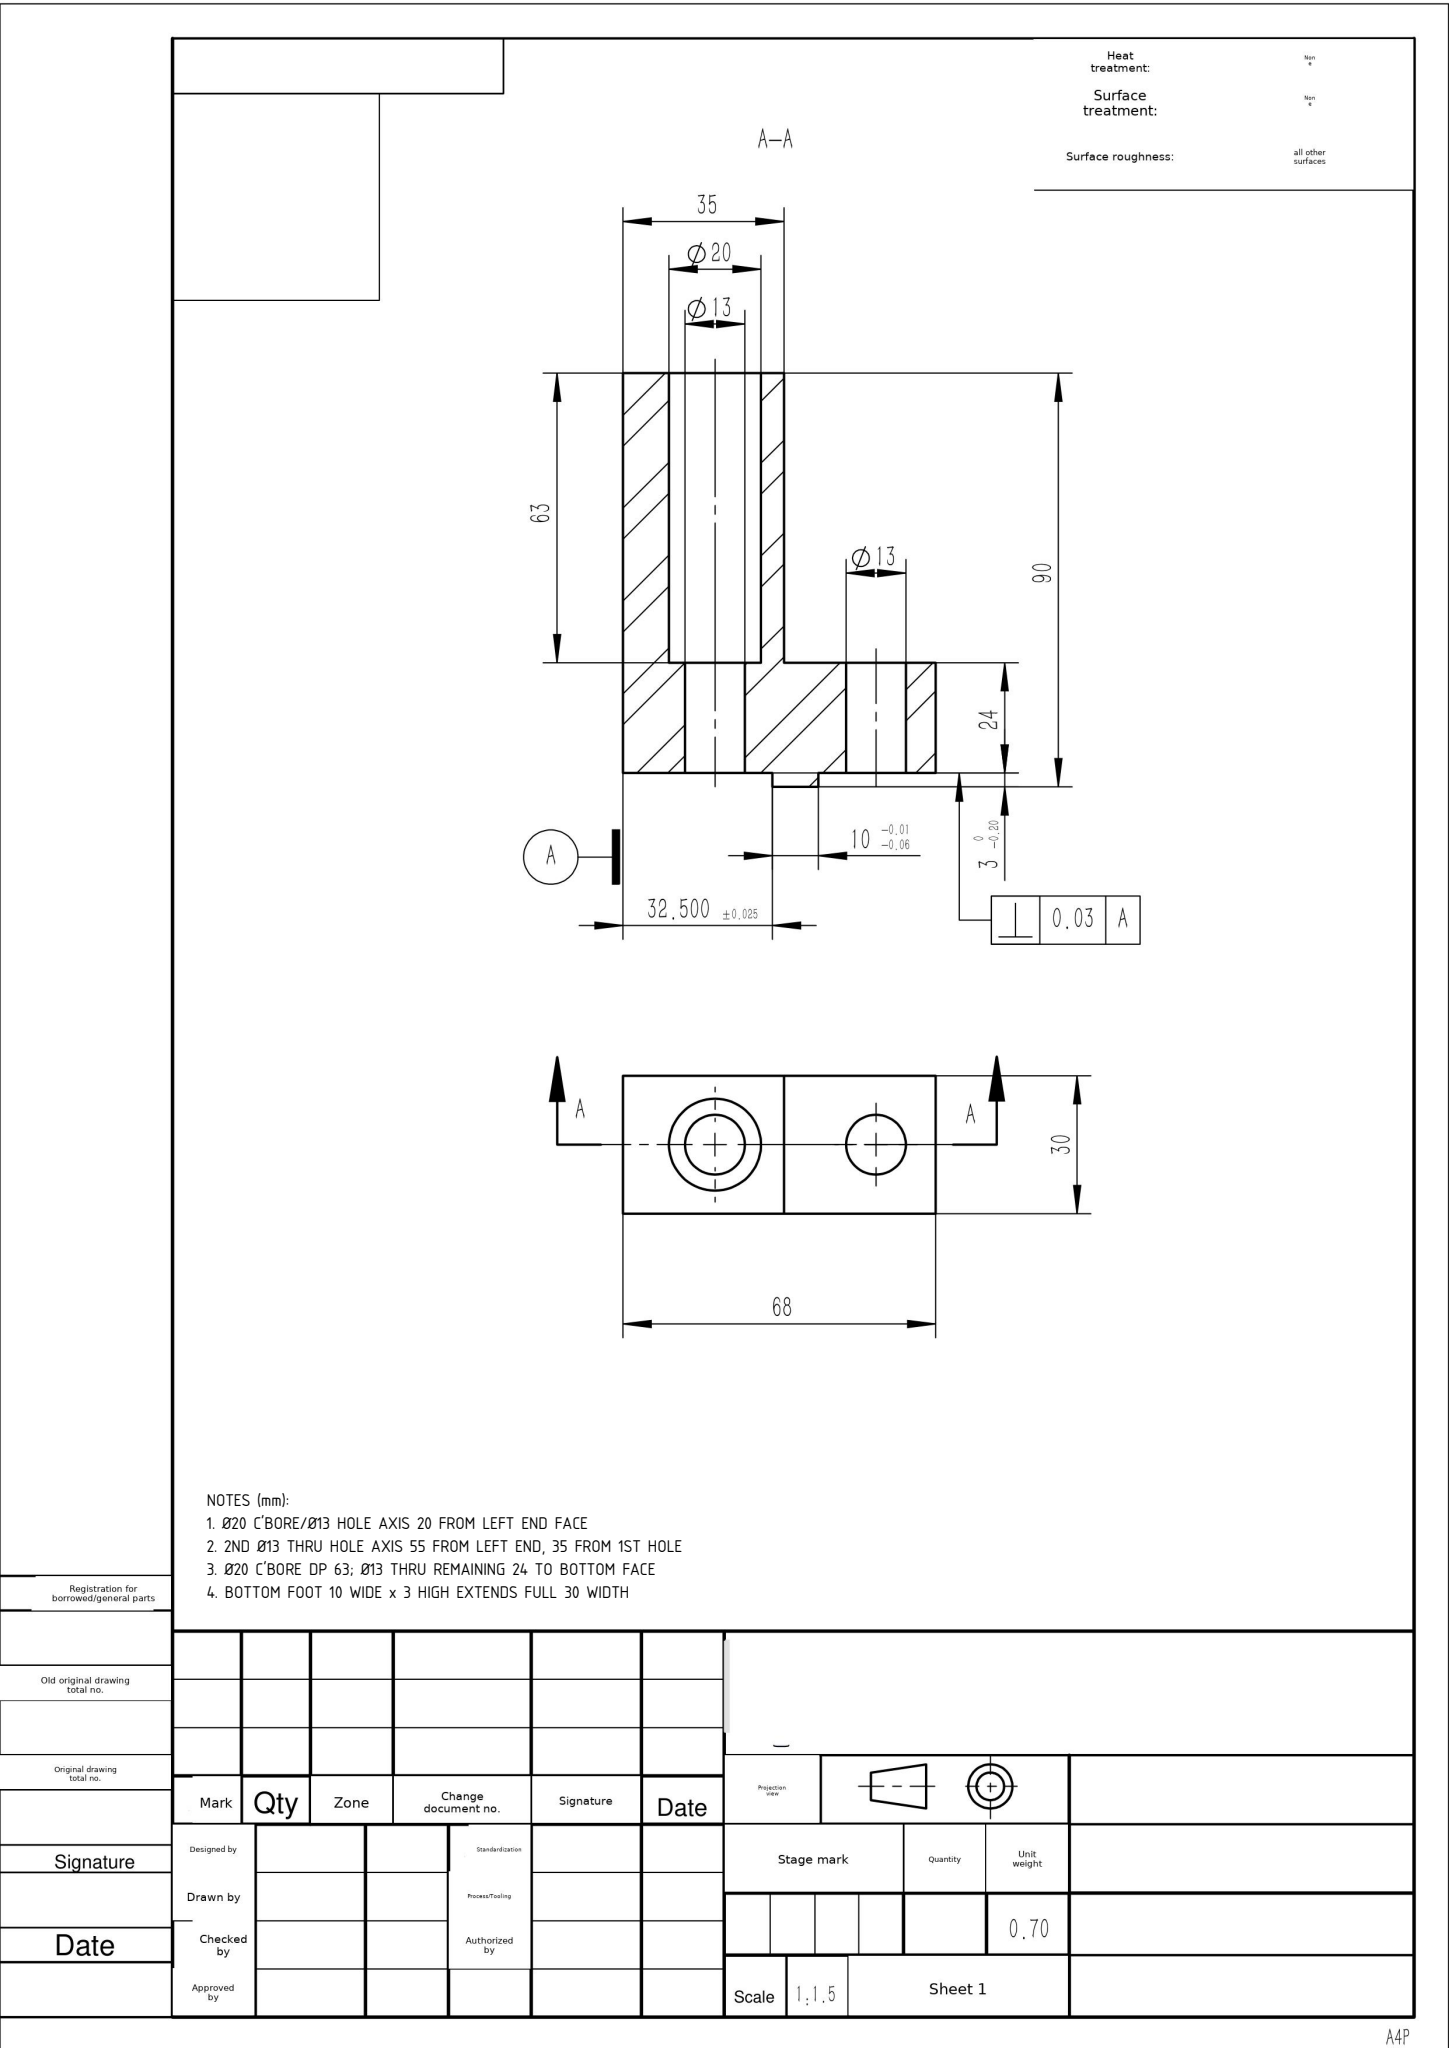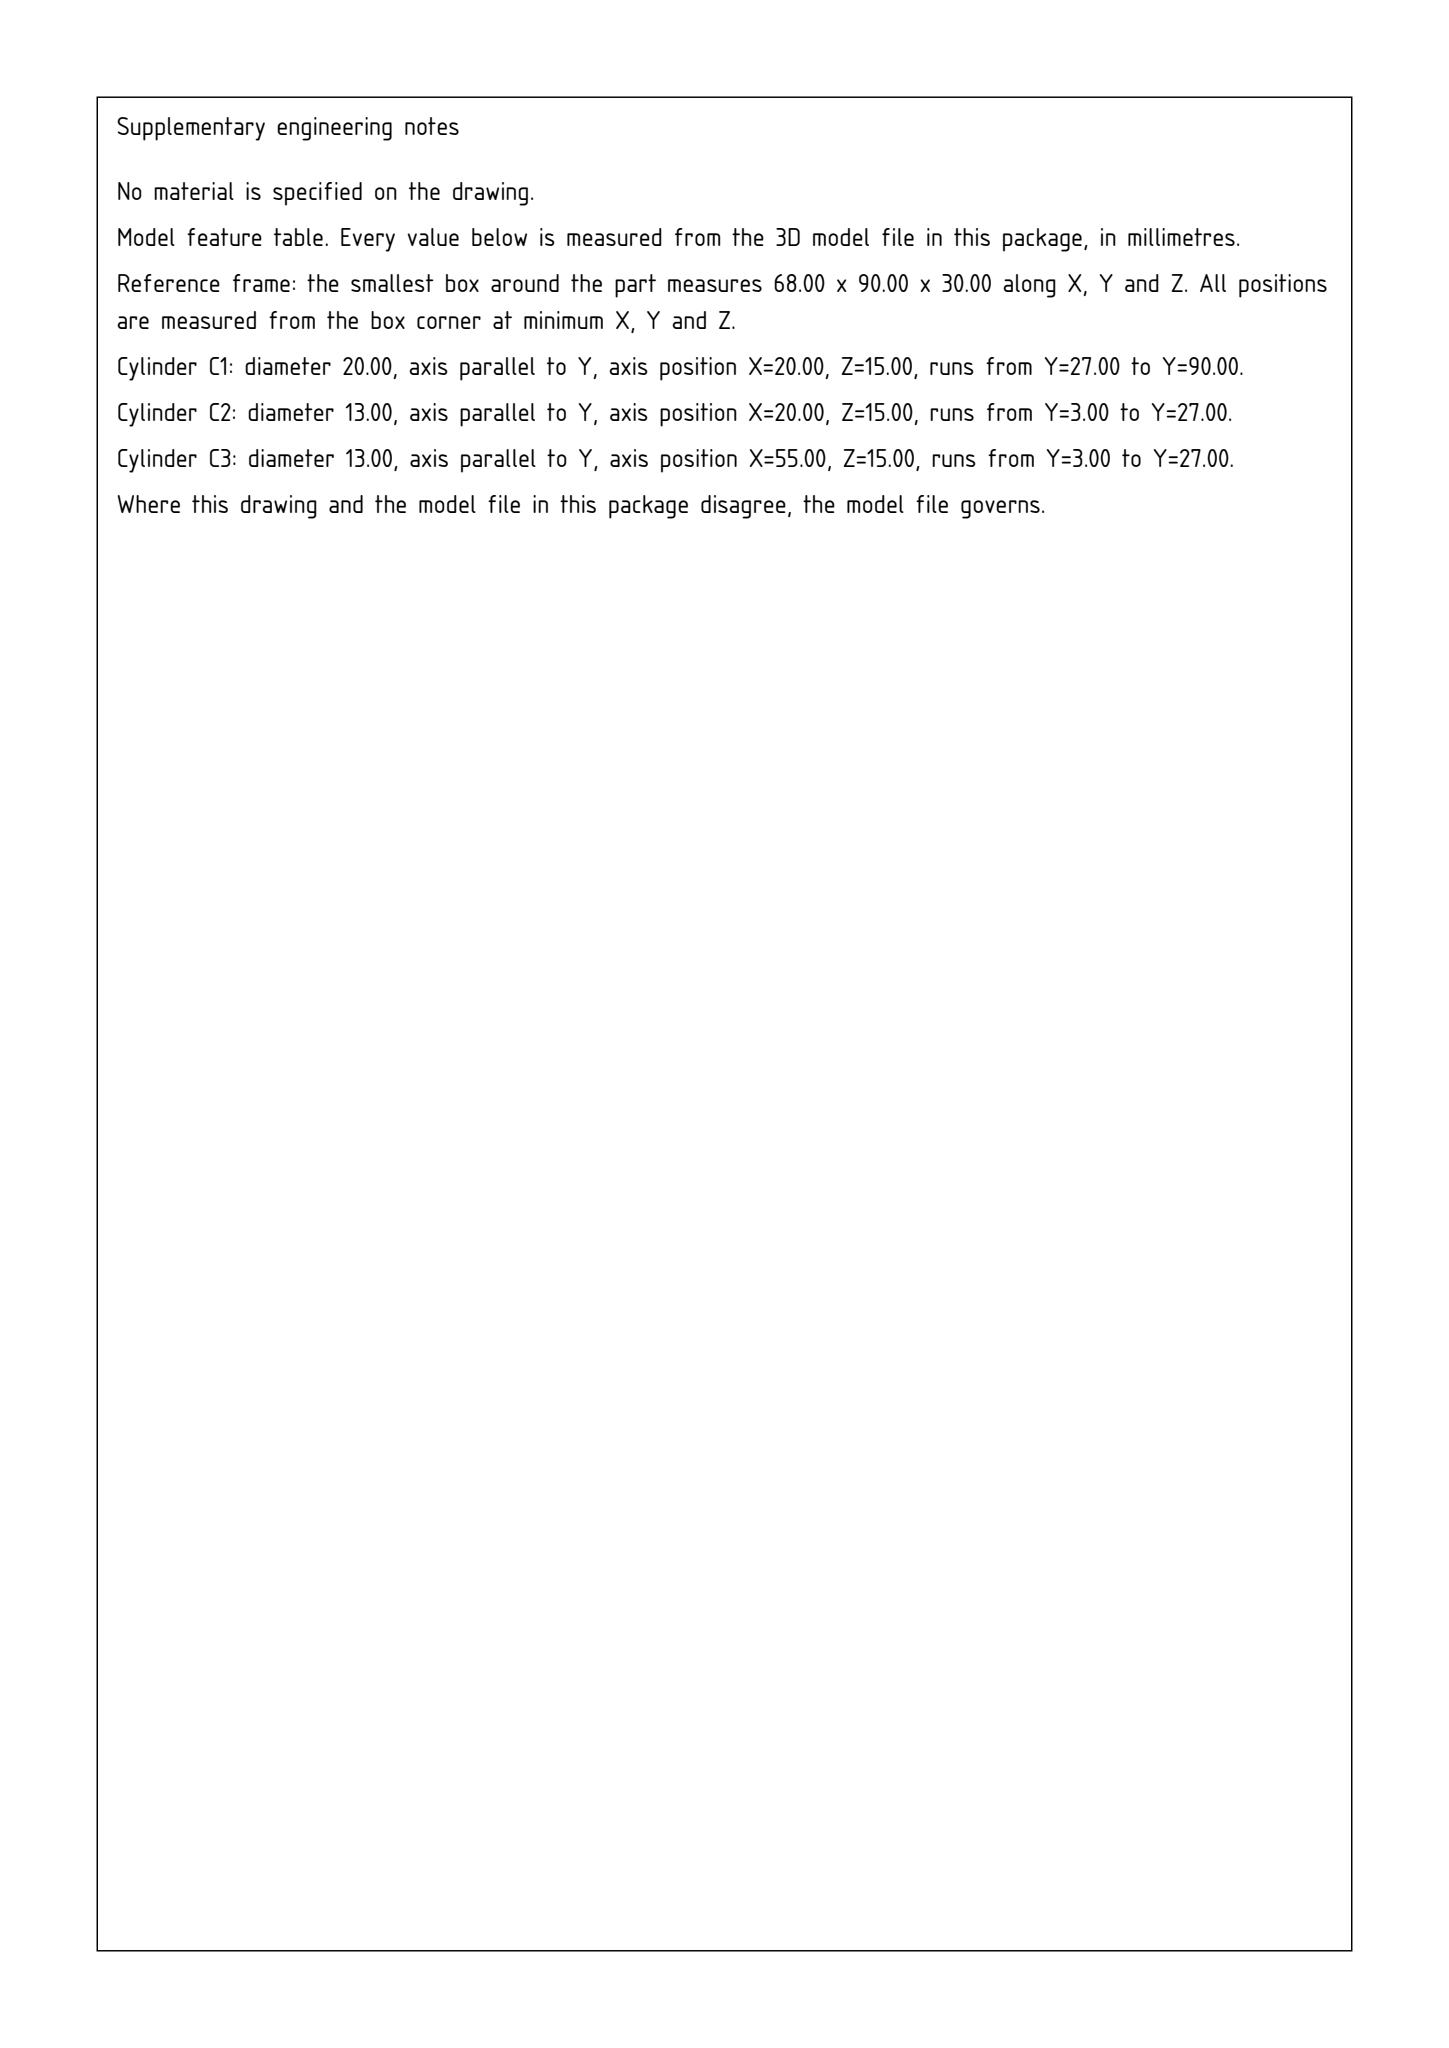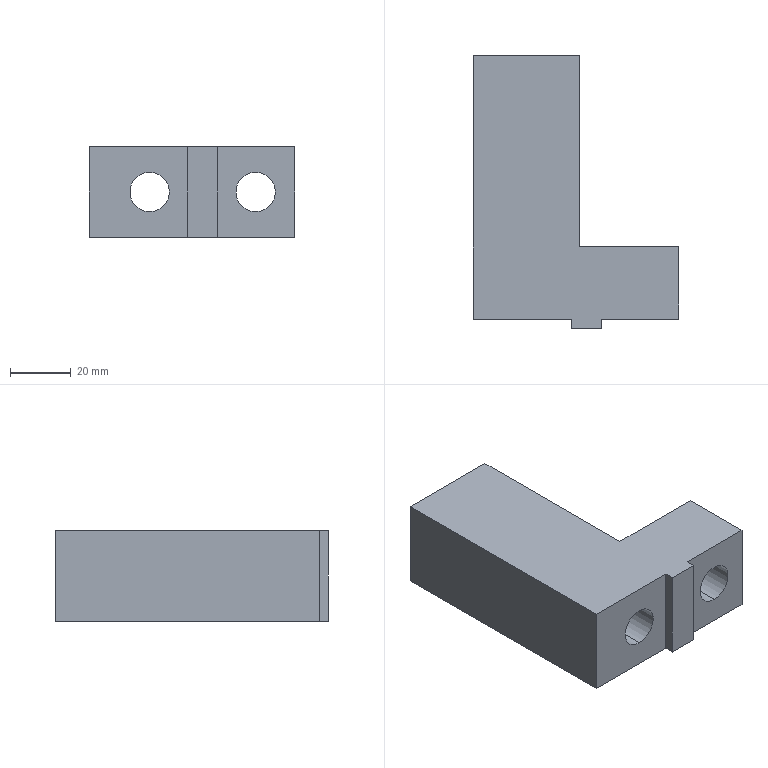Part | SolidWorks | mm | 1 solid | 19 faces | box 68 x 90 x 30 mm | volume 89847 mm3 | plane 13 | cylinder 6 | commonest cylinder face diameters 13 x4 20 x2
Drawing notes:
Ø20 C'BORE/Ø13 HOLE AXIS 20 FROM LEFT END FACE | from the solid: Ø20 & Ø13 cylinders, axis at x=20.0 (bbox x 0-68)
2ND Ø13 THRU HOLE AXIS 55 FROM LEFT END, 35 FROM 1ST HOLE | from the solid: Ø13 cylinder axis at x=55.0; 55-20=35 spacing
Ø20 C'BORE DP 63; Ø13 THRU REMAINING 24 TO BOTTOM FACE | from the solid: Ø20 L=63 (y 27-90), Ø13 L=24 (y 3-27) coaxial at x=20
BOTTOM FOOT 10 WIDE x 3 HIGH EXTENDS FULL 30 WIDTH | from the solid: x-planes 32.5 & 42.5, y-plane 3.0, z-planes 0.0 & 30.0 (bbox z=30)
build123d program:
from build123d import *

# Parameters (mm, degrees)
BOSS_EXTRUDE1_DEPTH = 15
SKETCH2_R           = 6.5
CUT_EXTRUDE1_DEPTH  = 114.794
SKETCH4_W           = 25.5
SKETCH4_H           = 3
SKETCH4_W_2         = 32.5
CUT_EXTRUDE3_DEPTH  = 117.722
SKETCH8_R           = 10
CUT_EXTRUDE6_DEPTH  = 63


with BuildPart() as part:
    # Sketch1 → Boss-Extrude1 (new, symmetric)
    with BuildSketch(Plane.XY):
        Polygon((0, 0), (0, 90), (35, 90), (35, 27), (68, 27), (68, 0), align=None)
    extrude(amount=BOSS_EXTRUDE1_DEPTH, both=True)

    # Sketch2 → Cut-Extrude1 (cut, through all)
    with BuildSketch(Plane(origin=(0, 90, 0), x_dir=(1, 0, 0), z_dir=(0, 1, 0))):
        with Locations(Location((20, 0, 0), (0, 0, 270))):
            Circle(SKETCH2_R)
        with Locations(Location((55, 0, 0), (0, 0, 270))):
            Circle(SKETCH2_R)
    extrude(amount=-CUT_EXTRUDE1_DEPTH, mode=Mode.SUBTRACT)

    # Sketch4 → Cut-Extrude3 (cut, through all)
    with BuildSketch(Plane.XY.offset(15)):
        with Locations((55.25, 1.5)):
            Rectangle(SKETCH4_W, SKETCH4_H)
        with Locations((16.25, 1.5)):
            Rectangle(SKETCH4_W_2, SKETCH4_H)
    extrude(amount=-CUT_EXTRUDE3_DEPTH, mode=Mode.SUBTRACT)

    # Sketch8 → Cut-Extrude6 (cut)
    with BuildSketch(Plane(origin=(0, 90, 0), x_dir=(1, 0, 0), z_dir=(0, 1, 0))):
        with Locations(Location((20, 0, 0), (0, 0, 270))):
            Circle(SKETCH8_R)
    extrude(amount=-CUT_EXTRUDE6_DEPTH, mode=Mode.SUBTRACT)


solid = part.part
STEP:
#1=CARTESIAN_POINT('',(20.,27.,-10.));
#2=VERTEX_POINT('',#1);
#3=CARTESIAN_POINT('',(20.,27.,10.));
#4=VERTEX_POINT('',#3);
#5=CARTESIAN_POINT('',(20.,27.,0.));
#6=DIRECTION('',(0.,1.,0.));
#7=DIRECTION('',(0.,0.,-1.));
#8=AXIS2_PLACEMENT_3D('',#5,#6,#7);
#9=CIRCLE('',#8,10.);
#10=EDGE_CURVE('',#2,#4,#9,.T.);
#11=ORIENTED_EDGE('',*,*,#10,.F.);
#12=CARTESIAN_POINT('',(20.,90.,-10.));
#13=VERTEX_POINT('',#12);
#14=CARTESIAN_POINT('',(20.,-1.284,-10.));
#15=DIRECTION('',(0.,1.,0.));
#16=VECTOR('',#15,1000.);
#17=LINE('',#14,#16);
#18=EDGE_CURVE('',#2,#13,#17,.T.);
#19=ORIENTED_EDGE('',*,*,#18,.T.);
#20=CARTESIAN_POINT('',(20.,90.,10.));
#21=VERTEX_POINT('',#20);
#22=CARTESIAN_POINT('',(20.,90.,0.));
#23=DIRECTION('',(0.,1.,0.));
#24=DIRECTION('',(0.,0.,1.));
#25=AXIS2_PLACEMENT_3D('',#22,#23,#24);
#26=CIRCLE('',#25,10.);
#27=EDGE_CURVE('',#13,#21,#26,.T.);
#28=ORIENTED_EDGE('',*,*,#27,.T.);
#29=CARTESIAN_POINT('',(20.,-1.284,10.));
#30=DIRECTION('',(0.,1.,0.));
#31=VECTOR('',#30,1000.);
#32=LINE('',#29,#31);
#33=EDGE_CURVE('',#4,#21,#32,.T.);
#34=ORIENTED_EDGE('',*,*,#33,.F.);
#35=EDGE_LOOP('',(#11,#19,#28,#34));
#36=FACE_OUTER_BOUND('',#35,.T.);
#37=CARTESIAN_POINT('',(20.,-1.284,0.));
#38=DIRECTION('',(0.,1.,0.));
#39=DIRECTION('',(0.,0.,1.));
#40=AXIS2_PLACEMENT_3D('',#37,#38,#39);
#41=CYLINDRICAL_SURFACE('',#40,10.);
#42=ADVANCED_FACE('',(#36),#41,.F.);
#43=CARTESIAN_POINT('',(55.,3.,6.5));
#44=VERTEX_POINT('',#43);
#45=CARTESIAN_POINT('',(55.,3.,-6.5));
#46=VERTEX_POINT('',#45);
#47=CARTESIAN_POINT('',(55.,3.,0.));
#48=DIRECTION('',(0.,-1.,0.));
#49=DIRECTION('',(-1.,-0.,0.));
#50=AXIS2_PLACEMENT_3D('',#47,#48,#49);
#51=CIRCLE('',#50,6.5);
#52=EDGE_CURVE('',#44,#46,#51,.T.);
#53=ORIENTED_EDGE('',*,*,#52,.T.);
#54=CARTESIAN_POINT('',(55.,27.,-6.5));
#55=VERTEX_POINT('',#54);
#56=CARTESIAN_POINT('',(55.,0.,-6.5));
#57=DIRECTION('',(0.,1.,0.));
#58=VECTOR('',#57,1000.);
#59=LINE('',#56,#58);
#60=EDGE_CURVE('',#46,#55,#59,.T.);
#61=ORIENTED_EDGE('',*,*,#60,.T.);
#62=CARTESIAN_POINT('',(55.,27.,6.5));
#63=VERTEX_POINT('',#62);
#64=CARTESIAN_POINT('',(55.,27.,0.));
#65=DIRECTION('',(0.,-1.,0.));
#66=DIRECTION('',(0.,0.,-1.));
#67=AXIS2_PLACEMENT_3D('',#64,#65,#66);
#68=CIRCLE('',#67,6.5);
#69=EDGE_CURVE('',#63,#55,#68,.T.);
#70=ORIENTED_EDGE('',*,*,#69,.F.);
#71=CARTESIAN_POINT('',(55.,0.,6.5));
#72=DIRECTION('',(0.,1.,0.));
#73=VECTOR('',#72,1000.);
#74=LINE('',#71,#73);
#75=EDGE_CURVE('',#44,#63,#74,.T.);
#76=ORIENTED_EDGE('',*,*,#75,.F.);
#77=EDGE_LOOP('',(#53,#61,#70,#76));
#78=FACE_OUTER_BOUND('',#77,.T.);
#79=CARTESIAN_POINT('',(55.,0.,0.));
#80=DIRECTION('',(0.,1.,0.));
#81=DIRECTION('',(0.,0.,1.));
#82=AXIS2_PLACEMENT_3D('',#79,#80,#81);
#83=CYLINDRICAL_SURFACE('',#82,6.5);
#84=ADVANCED_FACE('',(#78),#83,.F.);
#85=CARTESIAN_POINT('',(20.,3.,6.5));
#86=VERTEX_POINT('',#85);
#87=CARTESIAN_POINT('',(20.,3.,-6.5));
#88=VERTEX_POINT('',#87);
#89=CARTESIAN_POINT('',(20.,3.,0.));
#90=DIRECTION('',(0.,-1.,0.));
#91=DIRECTION('',(-1.,-0.,0.));
#92=AXIS2_PLACEMENT_3D('',#89,#90,#91);
#93=CIRCLE('',#92,6.5);
#94=EDGE_CURVE('',#86,#88,#93,.T.);
#95=ORIENTED_EDGE('',*,*,#94,.T.);
#96=CARTESIAN_POINT('',(20.,27.,-6.5));
#97=VERTEX_POINT('',#96);
#98=CARTESIAN_POINT('',(20.,0.,-6.5));
#99=DIRECTION('',(0.,1.,0.));
#100=VECTOR('',#99,1000.);
#101=LINE('',#98,#100);
#102=EDGE_CURVE('',#88,#97,#101,.T.);
#103=ORIENTED_EDGE('',*,*,#102,.T.);
#104=CARTESIAN_POINT('',(20.,27.,6.5));
#105=VERTEX_POINT('',#104);
#106=CARTESIAN_POINT('',(20.,27.,0.));
#107=DIRECTION('',(0.,1.,0.));
#108=DIRECTION('',(0.,0.,-1.));
#109=AXIS2_PLACEMENT_3D('',#106,#107,#108);
#110=CIRCLE('',#109,6.5);
#111=EDGE_CURVE('',#97,#105,#110,.T.);
#112=ORIENTED_EDGE('',*,*,#111,.T.);
#113=CARTESIAN_POINT('',(20.,0.,6.5));
#114=DIRECTION('',(0.,1.,0.));
#115=VECTOR('',#114,1000.);
#116=LINE('',#113,#115);
#117=EDGE_CURVE('',#86,#105,#116,.T.);
#118=ORIENTED_EDGE('',*,*,#117,.F.);
#119=EDGE_LOOP('',(#95,#103,#112,#118));
#120=FACE_OUTER_BOUND('',#119,.T.);
#121=CARTESIAN_POINT('',(20.,0.,0.));
#122=DIRECTION('',(0.,1.,0.));
#123=DIRECTION('',(0.,0.,1.));
#124=AXIS2_PLACEMENT_3D('',#121,#122,#123);
#125=CYLINDRICAL_SURFACE('',#124,6.5);
#126=ADVANCED_FACE('',(#120),#125,.F.);
#127=CARTESIAN_POINT('',(32.5,0.,15.));
#128=VERTEX_POINT('',#127);
#129=CARTESIAN_POINT('',(42.5,-0.,15.));
#130=VERTEX_POINT('',#129);
#131=CARTESIAN_POINT('',(68.,-0.,15.));
#132=DIRECTION('',(1.,-0.,0.));
#133=VECTOR('',#132,1000.);
#134=LINE('',#131,#133);
#135=EDGE_CURVE('',#128,#130,#134,.T.);
#136=ORIENTED_EDGE('',*,*,#135,.F.);
#137=CARTESIAN_POINT('',(32.5,0.,-15.));
#138=VERTEX_POINT('',#137);
#139=CARTESIAN_POINT('',(32.5,0.,-15.));
#140=DIRECTION('',(0.,0.,1.));
#141=VECTOR('',#140,1000.);
#142=LINE('',#139,#141);
#143=EDGE_CURVE('',#138,#128,#142,.T.);
#144=ORIENTED_EDGE('',*,*,#143,.F.);
#145=CARTESIAN_POINT('',(42.5,-0.,-15.));
#146=VERTEX_POINT('',#145);
#147=CARTESIAN_POINT('',(68.,-0.,-15.));
#148=DIRECTION('',(1.,-0.,0.));
#149=VECTOR('',#148,1000.);
#150=LINE('',#147,#149);
#151=EDGE_CURVE('',#138,#146,#150,.T.);
#152=ORIENTED_EDGE('',*,*,#151,.T.);
#153=CARTESIAN_POINT('',(42.5,-0.,-15.));
#154=DIRECTION('',(0.,0.,1.));
#155=VECTOR('',#154,1000.);
#156=LINE('',#153,#155);
#157=EDGE_CURVE('',#146,#130,#156,.T.);
#158=ORIENTED_EDGE('',*,*,#157,.T.);
#159=EDGE_LOOP('',(#136,#144,#152,#158));
#160=FACE_OUTER_BOUND('',#159,.T.);
#161=CARTESIAN_POINT('',(68.,-0.,15.));
#162=DIRECTION('',(0.,1.,0.));
#163=DIRECTION('',(-1.,0.,0.));
#164=AXIS2_PLACEMENT_3D('',#161,#162,#163);
#165=PLANE('',#164);
#166=ADVANCED_FACE('',(#160),#165,.F.);
#167=CARTESIAN_POINT('',(68.,3.,15.));
#168=VERTEX_POINT('',#167);
#169=CARTESIAN_POINT('',(68.,27.,15.));
#170=VERTEX_POINT('',#169);
#171=CARTESIAN_POINT('',(68.,27.,15.));
#172=DIRECTION('',(0.,1.,0.));
#173=VECTOR('',#172,1000.);
#174=LINE('',#171,#173);
#175=EDGE_CURVE('',#168,#170,#174,.T.);
#176=ORIENTED_EDGE('',*,*,#175,.F.);
#177=CARTESIAN_POINT('',(68.,3.,-15.));
#178=VERTEX_POINT('',#177);
#179=CARTESIAN_POINT('',(68.,3.,-15.));
#180=DIRECTION('',(0.,0.,1.));
#181=VECTOR('',#180,1000.);
#182=LINE('',#179,#181);
#183=EDGE_CURVE('',#178,#168,#182,.T.);
#184=ORIENTED_EDGE('',*,*,#183,.F.);
#185=CARTESIAN_POINT('',(68.,27.,-15.));
#186=VERTEX_POINT('',#185);
#187=CARTESIAN_POINT('',(68.,27.,-15.));
#188=DIRECTION('',(0.,1.,0.));
#189=VECTOR('',#188,1000.);
#190=LINE('',#187,#189);
#191=EDGE_CURVE('',#178,#186,#190,.T.);
#192=ORIENTED_EDGE('',*,*,#191,.T.);
#193=CARTESIAN_POINT('',(68.,27.,15.));
#194=DIRECTION('',(0.,0.,-1.));
#195=VECTOR('',#194,1000.);
#196=LINE('',#193,#195);
#197=EDGE_CURVE('',#170,#186,#196,.T.);
#198=ORIENTED_EDGE('',*,*,#197,.F.);
#199=EDGE_LOOP('',(#176,#184,#192,#198));
#200=FACE_OUTER_BOUND('',#199,.T.);
#201=CARTESIAN_POINT('',(68.,27.,15.));
#202=DIRECTION('',(-1.,0.,0.));
#203=DIRECTION('',(0.,0.,1.));
#204=AXIS2_PLACEMENT_3D('',#201,#202,#203);
#205=PLANE('',#204);
#206=ADVANCED_FACE('',(#200),#205,.F.);
#207=ORIENTED_EDGE('',*,*,#69,.T.);
#208=CARTESIAN_POINT('',(55.,27.,0.));
#209=DIRECTION('',(0.,-1.,0.));
#210=DIRECTION('',(0.,0.,-1.));
#211=AXIS2_PLACEMENT_3D('',#208,#209,#210);
#212=CIRCLE('',#211,6.5);
#213=EDGE_CURVE('',#55,#63,#212,.T.);
#214=ORIENTED_EDGE('',*,*,#213,.T.);
#215=EDGE_LOOP('',(#207,#214));
#216=FACE_BOUND('',#215,.T.);
#217=CARTESIAN_POINT('',(35.,27.,-15.));
#218=VERTEX_POINT('',#217);
#219=CARTESIAN_POINT('',(35.,27.,-15.));
#220=DIRECTION('',(-1.,0.,0.));
#221=VECTOR('',#220,1000.);
#222=LINE('',#219,#221);
#223=EDGE_CURVE('',#186,#218,#222,.T.);
#224=ORIENTED_EDGE('',*,*,#223,.T.);
#225=CARTESIAN_POINT('',(35.,27.,15.));
#226=VERTEX_POINT('',#225);
#227=CARTESIAN_POINT('',(35.,27.,15.));
#228=DIRECTION('',(0.,0.,-1.));
#229=VECTOR('',#228,1000.);
#230=LINE('',#227,#229);
#231=EDGE_CURVE('',#226,#218,#230,.T.);
#232=ORIENTED_EDGE('',*,*,#231,.F.);
#233=CARTESIAN_POINT('',(35.,27.,15.));
#234=DIRECTION('',(-1.,0.,0.));
#235=VECTOR('',#234,1000.);
#236=LINE('',#233,#235);
#237=EDGE_CURVE('',#170,#226,#236,.T.);
#238=ORIENTED_EDGE('',*,*,#237,.F.);
#239=ORIENTED_EDGE('',*,*,#197,.T.);
#240=EDGE_LOOP('',(#224,#232,#238,#239));
#241=FACE_OUTER_BOUND('',#240,.T.);
#242=CARTESIAN_POINT('',(35.,27.,15.));
#243=DIRECTION('',(0.,-1.,0.));
#244=DIRECTION('',(0.,0.,-1.));
#245=AXIS2_PLACEMENT_3D('',#242,#243,#244);
#246=PLANE('',#245);
#247=ADVANCED_FACE('',(#216,#241),#246,.F.);
#248=CARTESIAN_POINT('',(35.,90.,-15.));
#249=VERTEX_POINT('',#248);
#250=CARTESIAN_POINT('',(35.,90.,-15.));
#251=DIRECTION('',(-0.,1.,0.));
#252=VECTOR('',#251,1000.);
#253=LINE('',#250,#252);
#254=EDGE_CURVE('',#218,#249,#253,.T.);
#255=ORIENTED_EDGE('',*,*,#254,.T.);
#256=CARTESIAN_POINT('',(35.,90.,15.));
#257=VERTEX_POINT('',#256);
#258=CARTESIAN_POINT('',(35.,90.,15.));
#259=DIRECTION('',(0.,0.,-1.));
#260=VECTOR('',#259,1000.);
#261=LINE('',#258,#260);
#262=EDGE_CURVE('',#257,#249,#261,.T.);
#263=ORIENTED_EDGE('',*,*,#262,.F.);
#264=CARTESIAN_POINT('',(35.,90.,15.));
#265=DIRECTION('',(-0.,1.,0.));
#266=VECTOR('',#265,1000.);
#267=LINE('',#264,#266);
#268=EDGE_CURVE('',#226,#257,#267,.T.);
#269=ORIENTED_EDGE('',*,*,#268,.F.);
#270=ORIENTED_EDGE('',*,*,#231,.T.);
#271=EDGE_LOOP('',(#255,#263,#269,#270));
#272=FACE_OUTER_BOUND('',#271,.T.);
#273=CARTESIAN_POINT('',(35.,90.,15.));
#274=DIRECTION('',(-1.,-0.,0.));
#275=DIRECTION('',(0.,-1.,0.));
#276=AXIS2_PLACEMENT_3D('',#273,#274,#275);
#277=PLANE('',#276);
#278=ADVANCED_FACE('',(#272),#277,.F.);
#279=CARTESIAN_POINT('',(20.,90.,0.));
#280=DIRECTION('',(0.,1.,0.));
#281=DIRECTION('',(0.,0.,1.));
#282=AXIS2_PLACEMENT_3D('',#279,#280,#281);
#283=CIRCLE('',#282,10.);
#284=EDGE_CURVE('',#21,#13,#283,.T.);
#285=ORIENTED_EDGE('',*,*,#284,.F.);
#286=ORIENTED_EDGE('',*,*,#27,.F.);
#287=EDGE_LOOP('',(#285,#286));
#288=FACE_BOUND('',#287,.T.);
#289=CARTESIAN_POINT('',(0.,90.,-15.));
#290=VERTEX_POINT('',#289);
#291=CARTESIAN_POINT('',(0.,90.,-15.));
#292=DIRECTION('',(-1.,0.,0.));
#293=VECTOR('',#292,1000.);
#294=LINE('',#291,#293);
#295=EDGE_CURVE('',#249,#290,#294,.T.);
#296=ORIENTED_EDGE('',*,*,#295,.T.);
#297=CARTESIAN_POINT('',(0.,90.,15.));
#298=VERTEX_POINT('',#297);
#299=CARTESIAN_POINT('',(0.,90.,15.));
#300=DIRECTION('',(0.,0.,-1.));
#301=VECTOR('',#300,1000.);
#302=LINE('',#299,#301);
#303=EDGE_CURVE('',#298,#290,#302,.T.);
#304=ORIENTED_EDGE('',*,*,#303,.F.);
#305=CARTESIAN_POINT('',(0.,90.,15.));
#306=DIRECTION('',(-1.,0.,0.));
#307=VECTOR('',#306,1000.);
#308=LINE('',#305,#307);
#309=EDGE_CURVE('',#257,#298,#308,.T.);
#310=ORIENTED_EDGE('',*,*,#309,.F.);
#311=ORIENTED_EDGE('',*,*,#262,.T.);
#312=EDGE_LOOP('',(#296,#304,#310,#311));
#313=FACE_OUTER_BOUND('',#312,.T.);
#314=CARTESIAN_POINT('',(0.,90.,15.));
#315=DIRECTION('',(0.,-1.,0.));
#316=DIRECTION('',(0.,0.,-1.));
#317=AXIS2_PLACEMENT_3D('',#314,#315,#316);
#318=PLANE('',#317);
#319=ADVANCED_FACE('',(#288,#313),#318,.F.);
#320=CARTESIAN_POINT('',(0.,3.,-15.));
#321=VERTEX_POINT('',#320);
#322=CARTESIAN_POINT('',(0.,0.,-15.));
#323=DIRECTION('',(0.,-1.,0.));
#324=VECTOR('',#323,1000.);
#325=LINE('',#322,#324);
#326=EDGE_CURVE('',#290,#321,#325,.T.);
#327=ORIENTED_EDGE('',*,*,#326,.T.);
#328=CARTESIAN_POINT('',(0.,3.,15.));
#329=VERTEX_POINT('',#328);
#330=CARTESIAN_POINT('',(0.,3.,-15.));
#331=DIRECTION('',(0.,0.,1.));
#332=VECTOR('',#331,1000.);
#333=LINE('',#330,#332);
#334=EDGE_CURVE('',#321,#329,#333,.T.);
#335=ORIENTED_EDGE('',*,*,#334,.T.);
#336=CARTESIAN_POINT('',(0.,0.,15.));
#337=DIRECTION('',(0.,-1.,0.));
#338=VECTOR('',#337,1000.);
#339=LINE('',#336,#338);
#340=EDGE_CURVE('',#298,#329,#339,.T.);
#341=ORIENTED_EDGE('',*,*,#340,.F.);
#342=ORIENTED_EDGE('',*,*,#303,.T.);
#343=EDGE_LOOP('',(#327,#335,#341,#342));
#344=FACE_OUTER_BOUND('',#343,.T.);
#345=CARTESIAN_POINT('',(0.,0.,15.));
#346=DIRECTION('',(1.,0.,0.));
#347=DIRECTION('',(0.,0.,-1.));
#348=AXIS2_PLACEMENT_3D('',#345,#346,#347);
#349=PLANE('',#348);
#350=ADVANCED_FACE('',(#344),#349,.F.);
#351=ORIENTED_EDGE('',*,*,#340,.T.);
#352=CARTESIAN_POINT('',(32.5,3.,15.));
#353=VERTEX_POINT('',#352);
#354=CARTESIAN_POINT('',(0.,3.,15.));
#355=DIRECTION('',(-1.,-0.,0.));
#356=VECTOR('',#355,1000.);
#357=LINE('',#354,#356);
#358=EDGE_CURVE('',#353,#329,#357,.T.);
#359=ORIENTED_EDGE('',*,*,#358,.F.);
#360=CARTESIAN_POINT('',(32.5,0.,15.));
#361=DIRECTION('',(0.,1.,0.));
#362=VECTOR('',#361,1000.);
#363=LINE('',#360,#362);
#364=EDGE_CURVE('',#128,#353,#363,.T.);
#365=ORIENTED_EDGE('',*,*,#364,.F.);
#366=ORIENTED_EDGE('',*,*,#135,.T.);
#367=CARTESIAN_POINT('',(42.5,3.,15.));
#368=VERTEX_POINT('',#367);
#369=CARTESIAN_POINT('',(42.5,-0.,15.));
#370=DIRECTION('',(0.,-1.,0.));
#371=VECTOR('',#370,1000.);
#372=LINE('',#369,#371);
#373=EDGE_CURVE('',#368,#130,#372,.T.);
#374=ORIENTED_EDGE('',*,*,#373,.F.);
#375=CARTESIAN_POINT('',(68.,3.,15.));
#376=DIRECTION('',(-1.,-0.,0.));
#377=VECTOR('',#376,1000.);
#378=LINE('',#375,#377);
#379=EDGE_CURVE('',#168,#368,#378,.T.);
#380=ORIENTED_EDGE('',*,*,#379,.F.);
#381=ORIENTED_EDGE('',*,*,#175,.T.);
#382=ORIENTED_EDGE('',*,*,#237,.T.);
#383=ORIENTED_EDGE('',*,*,#268,.T.);
#384=ORIENTED_EDGE('',*,*,#309,.T.);
#385=EDGE_LOOP('',(#351,#359,#365,#366,#374,#380,#381,#382,#383,#384));
#386=FACE_OUTER_BOUND('',#385,.T.);
#387=CARTESIAN_POINT('',(0.,0.,15.));
#388=DIRECTION('',(0.,0.,-1.));
#389=DIRECTION('',(-1.,0.,0.));
#390=AXIS2_PLACEMENT_3D('',#387,#388,#389);
#391=PLANE('',#390);
#392=ADVANCED_FACE('',(#386),#391,.F.);
#393=CARTESIAN_POINT('',(32.5,3.,-15.));
#394=VERTEX_POINT('',#393);
#395=CARTESIAN_POINT('',(0.,3.,-15.));
#396=DIRECTION('',(-1.,-0.,0.));
#397=VECTOR('',#396,1000.);
#398=LINE('',#395,#397);
#399=EDGE_CURVE('',#394,#321,#398,.T.);
#400=ORIENTED_EDGE('',*,*,#399,.T.);
#401=ORIENTED_EDGE('',*,*,#326,.F.);
#402=ORIENTED_EDGE('',*,*,#295,.F.);
#403=ORIENTED_EDGE('',*,*,#254,.F.);
#404=ORIENTED_EDGE('',*,*,#223,.F.);
#405=ORIENTED_EDGE('',*,*,#191,.F.);
#406=CARTESIAN_POINT('',(42.5,3.,-15.));
#407=VERTEX_POINT('',#406);
#408=CARTESIAN_POINT('',(68.,3.,-15.));
#409=DIRECTION('',(-1.,-0.,0.));
#410=VECTOR('',#409,1000.);
#411=LINE('',#408,#410);
#412=EDGE_CURVE('',#178,#407,#411,.T.);
#413=ORIENTED_EDGE('',*,*,#412,.T.);
#414=CARTESIAN_POINT('',(42.5,-0.,-15.));
#415=DIRECTION('',(0.,-1.,0.));
#416=VECTOR('',#415,1000.);
#417=LINE('',#414,#416);
#418=EDGE_CURVE('',#407,#146,#417,.T.);
#419=ORIENTED_EDGE('',*,*,#418,.T.);
#420=ORIENTED_EDGE('',*,*,#151,.F.);
#421=CARTESIAN_POINT('',(32.5,0.,-15.));
#422=DIRECTION('',(0.,1.,0.));
#423=VECTOR('',#422,1000.);
#424=LINE('',#421,#423);
#425=EDGE_CURVE('',#138,#394,#424,.T.);
#426=ORIENTED_EDGE('',*,*,#425,.T.);
#427=EDGE_LOOP('',(#400,#401,#402,#403,#404,#405,#413,#419,#420,#426));
#428=FACE_OUTER_BOUND('',#427,.T.);
#429=CARTESIAN_POINT('',(0.,0.,-15.));
#430=DIRECTION('',(0.,0.,-1.));
#431=DIRECTION('',(-1.,0.,0.));
#432=AXIS2_PLACEMENT_3D('',#429,#430,#431);
#433=PLANE('',#432);
#434=ADVANCED_FACE('',(#428),#433,.T.);
#435=ORIENTED_EDGE('',*,*,#102,.F.);
#436=CARTESIAN_POINT('',(20.,3.,0.));
#437=DIRECTION('',(0.,-1.,0.));
#438=DIRECTION('',(-1.,-0.,0.));
#439=AXIS2_PLACEMENT_3D('',#436,#437,#438);
#440=CIRCLE('',#439,6.5);
#441=EDGE_CURVE('',#88,#86,#440,.T.);
#442=ORIENTED_EDGE('',*,*,#441,.T.);
#443=ORIENTED_EDGE('',*,*,#117,.T.);
#444=CARTESIAN_POINT('',(20.,27.,0.));
#445=DIRECTION('',(0.,1.,0.));
#446=DIRECTION('',(0.,0.,-1.));
#447=AXIS2_PLACEMENT_3D('',#444,#445,#446);
#448=CIRCLE('',#447,6.5);
#449=EDGE_CURVE('',#105,#97,#448,.T.);
#450=ORIENTED_EDGE('',*,*,#449,.T.);
#451=EDGE_LOOP('',(#435,#442,#443,#450));
#452=FACE_OUTER_BOUND('',#451,.T.);
#453=CARTESIAN_POINT('',(20.,0.,0.));
#454=DIRECTION('',(0.,1.,0.));
#455=DIRECTION('',(0.,0.,1.));
#456=AXIS2_PLACEMENT_3D('',#453,#454,#455);
#457=CYLINDRICAL_SURFACE('',#456,6.5);
#458=ADVANCED_FACE('',(#452),#457,.F.);
#459=ORIENTED_EDGE('',*,*,#60,.F.);
#460=CARTESIAN_POINT('',(55.,3.,0.));
#461=DIRECTION('',(0.,-1.,0.));
#462=DIRECTION('',(-1.,-0.,0.));
#463=AXIS2_PLACEMENT_3D('',#460,#461,#462);
#464=CIRCLE('',#463,6.5);
#465=EDGE_CURVE('',#46,#44,#464,.T.);
#466=ORIENTED_EDGE('',*,*,#465,.T.);
#467=ORIENTED_EDGE('',*,*,#75,.T.);
#468=ORIENTED_EDGE('',*,*,#213,.F.);
#469=EDGE_LOOP('',(#459,#466,#467,#468));
#470=FACE_OUTER_BOUND('',#469,.T.);
#471=CARTESIAN_POINT('',(55.,0.,0.));
#472=DIRECTION('',(0.,1.,0.));
#473=DIRECTION('',(0.,0.,1.));
#474=AXIS2_PLACEMENT_3D('',#471,#472,#473);
#475=CYLINDRICAL_SURFACE('',#474,6.5);
#476=ADVANCED_FACE('',(#470),#475,.F.);
#477=ORIENTED_EDGE('',*,*,#379,.T.);
#478=CARTESIAN_POINT('',(42.5,3.,-15.));
#479=DIRECTION('',(0.,0.,1.));
#480=VECTOR('',#479,1000.);
#481=LINE('',#478,#480);
#482=EDGE_CURVE('',#407,#368,#481,.T.);
#483=ORIENTED_EDGE('',*,*,#482,.F.);
#484=ORIENTED_EDGE('',*,*,#412,.F.);
#485=ORIENTED_EDGE('',*,*,#183,.T.);
#486=EDGE_LOOP('',(#477,#483,#484,#485));
#487=FACE_OUTER_BOUND('',#486,.T.);
#488=ORIENTED_EDGE('',*,*,#52,.F.);
#489=ORIENTED_EDGE('',*,*,#465,.F.);
#490=EDGE_LOOP('',(#488,#489));
#491=FACE_BOUND('',#490,.T.);
#492=CARTESIAN_POINT('',(68.,3.,-15.));
#493=DIRECTION('',(-0.,1.,0.));
#494=DIRECTION('',(-1.,-0.,0.));
#495=AXIS2_PLACEMENT_3D('',#492,#493,#494);
#496=PLANE('',#495);
#497=ADVANCED_FACE('',(#487,#491),#496,.F.);
#498=ORIENTED_EDGE('',*,*,#373,.T.);
#499=ORIENTED_EDGE('',*,*,#157,.F.);
#500=ORIENTED_EDGE('',*,*,#418,.F.);
#501=ORIENTED_EDGE('',*,*,#482,.T.);
#502=EDGE_LOOP('',(#498,#499,#500,#501));
#503=FACE_OUTER_BOUND('',#502,.T.);
#504=CARTESIAN_POINT('',(42.5,-0.,-15.));
#505=DIRECTION('',(-1.,0.,0.));
#506=DIRECTION('',(0.,0.,1.));
#507=AXIS2_PLACEMENT_3D('',#504,#505,#506);
#508=PLANE('',#507);
#509=ADVANCED_FACE('',(#503),#508,.F.);
#510=ORIENTED_EDGE('',*,*,#358,.T.);
#511=ORIENTED_EDGE('',*,*,#334,.F.);
#512=ORIENTED_EDGE('',*,*,#399,.F.);
#513=CARTESIAN_POINT('',(32.5,3.,-15.));
#514=DIRECTION('',(0.,0.,1.));
#515=VECTOR('',#514,1000.);
#516=LINE('',#513,#515);
#517=EDGE_CURVE('',#394,#353,#516,.T.);
#518=ORIENTED_EDGE('',*,*,#517,.T.);
#519=EDGE_LOOP('',(#510,#511,#512,#518));
#520=FACE_OUTER_BOUND('',#519,.T.);
#521=ORIENTED_EDGE('',*,*,#94,.F.);
#522=ORIENTED_EDGE('',*,*,#441,.F.);
#523=EDGE_LOOP('',(#521,#522));
#524=FACE_BOUND('',#523,.T.);
#525=CARTESIAN_POINT('',(0.,3.,-15.));
#526=DIRECTION('',(-0.,1.,0.));
#527=DIRECTION('',(-1.,-0.,0.));
#528=AXIS2_PLACEMENT_3D('',#525,#526,#527);
#529=PLANE('',#528);
#530=ADVANCED_FACE('',(#520,#524),#529,.F.);
#531=ORIENTED_EDGE('',*,*,#364,.T.);
#532=ORIENTED_EDGE('',*,*,#517,.F.);
#533=ORIENTED_EDGE('',*,*,#425,.F.);
#534=ORIENTED_EDGE('',*,*,#143,.T.);
#535=EDGE_LOOP('',(#531,#532,#533,#534));
#536=FACE_OUTER_BOUND('',#535,.T.);
#537=CARTESIAN_POINT('',(32.5,0.,-15.));
#538=DIRECTION('',(1.,0.,0.));
#539=DIRECTION('',(0.,0.,-1.));
#540=AXIS2_PLACEMENT_3D('',#537,#538,#539);
#541=PLANE('',#540);
#542=ADVANCED_FACE('',(#536),#541,.F.);
#543=CARTESIAN_POINT('',(20.,27.,0.));
#544=DIRECTION('',(0.,1.,0.));
#545=DIRECTION('',(0.,0.,-1.));
#546=AXIS2_PLACEMENT_3D('',#543,#544,#545);
#547=CIRCLE('',#546,10.);
#548=EDGE_CURVE('',#4,#2,#547,.T.);
#549=ORIENTED_EDGE('',*,*,#548,.T.);
#550=ORIENTED_EDGE('',*,*,#10,.T.);
#551=EDGE_LOOP('',(#549,#550));
#552=FACE_OUTER_BOUND('',#551,.T.);
#553=ORIENTED_EDGE('',*,*,#449,.F.);
#554=ORIENTED_EDGE('',*,*,#111,.F.);
#555=EDGE_LOOP('',(#553,#554));
#556=FACE_BOUND('',#555,.T.);
#557=CARTESIAN_POINT('',(35.,27.,15.));
#558=DIRECTION('',(0.,-1.,0.));
#559=DIRECTION('',(0.,0.,-1.));
#560=AXIS2_PLACEMENT_3D('',#557,#558,#559);
#561=PLANE('',#560);
#562=ADVANCED_FACE('',(#552,#556),#561,.F.);
#563=ORIENTED_EDGE('',*,*,#18,.F.);
#564=ORIENTED_EDGE('',*,*,#548,.F.);
#565=ORIENTED_EDGE('',*,*,#33,.T.);
#566=ORIENTED_EDGE('',*,*,#284,.T.);
#567=EDGE_LOOP('',(#563,#564,#565,#566));
#568=FACE_OUTER_BOUND('',#567,.T.);
#569=CARTESIAN_POINT('',(20.,-1.284,0.));
#570=DIRECTION('',(0.,1.,0.));
#571=DIRECTION('',(0.,0.,1.));
#572=AXIS2_PLACEMENT_3D('',#569,#570,#571);
#573=CYLINDRICAL_SURFACE('',#572,10.);
#574=ADVANCED_FACE('',(#568),#573,.F.);
#575=CLOSED_SHELL('',(#42,#84,#126,#166,#206,#247,#278,#319,#350,#392,#434,#458,#476,#497,#509,#530,#542,#562,#574));
#576=MANIFOLD_SOLID_BREP('',#575);
#577=CARTESIAN_POINT('',(0.,0.,0.));
#578=DIRECTION('',(0.,0.,1.));
#579=DIRECTION('',(1.,0.,0.));
#580=AXIS2_PLACEMENT_3D('',#577,#578,#579);
#581=(LENGTH_UNIT()NAMED_UNIT(*)SI_UNIT(.MILLI.,.METRE.));
#582=UNCERTAINTY_MEASURE_WITH_UNIT(LENGTH_MEASURE(0.00001),#581,'','');
#583=(NAMED_UNIT(*)PLANE_ANGLE_UNIT()SI_UNIT($,.RADIAN.));
#584=(NAMED_UNIT(*)SI_UNIT($,.STERADIAN.)SOLID_ANGLE_UNIT());
#585=(GEOMETRIC_REPRESENTATION_CONTEXT(3)GLOBAL_UNCERTAINTY_ASSIGNED_CONTEXT((#582))GLOBAL_UNIT_ASSIGNED_CONTEXT((#581,#583,#584))REPRESENTATION_CONTEXT('',''));
#586=ADVANCED_BREP_SHAPE_REPRESENTATION('',(#576,#580),#585);